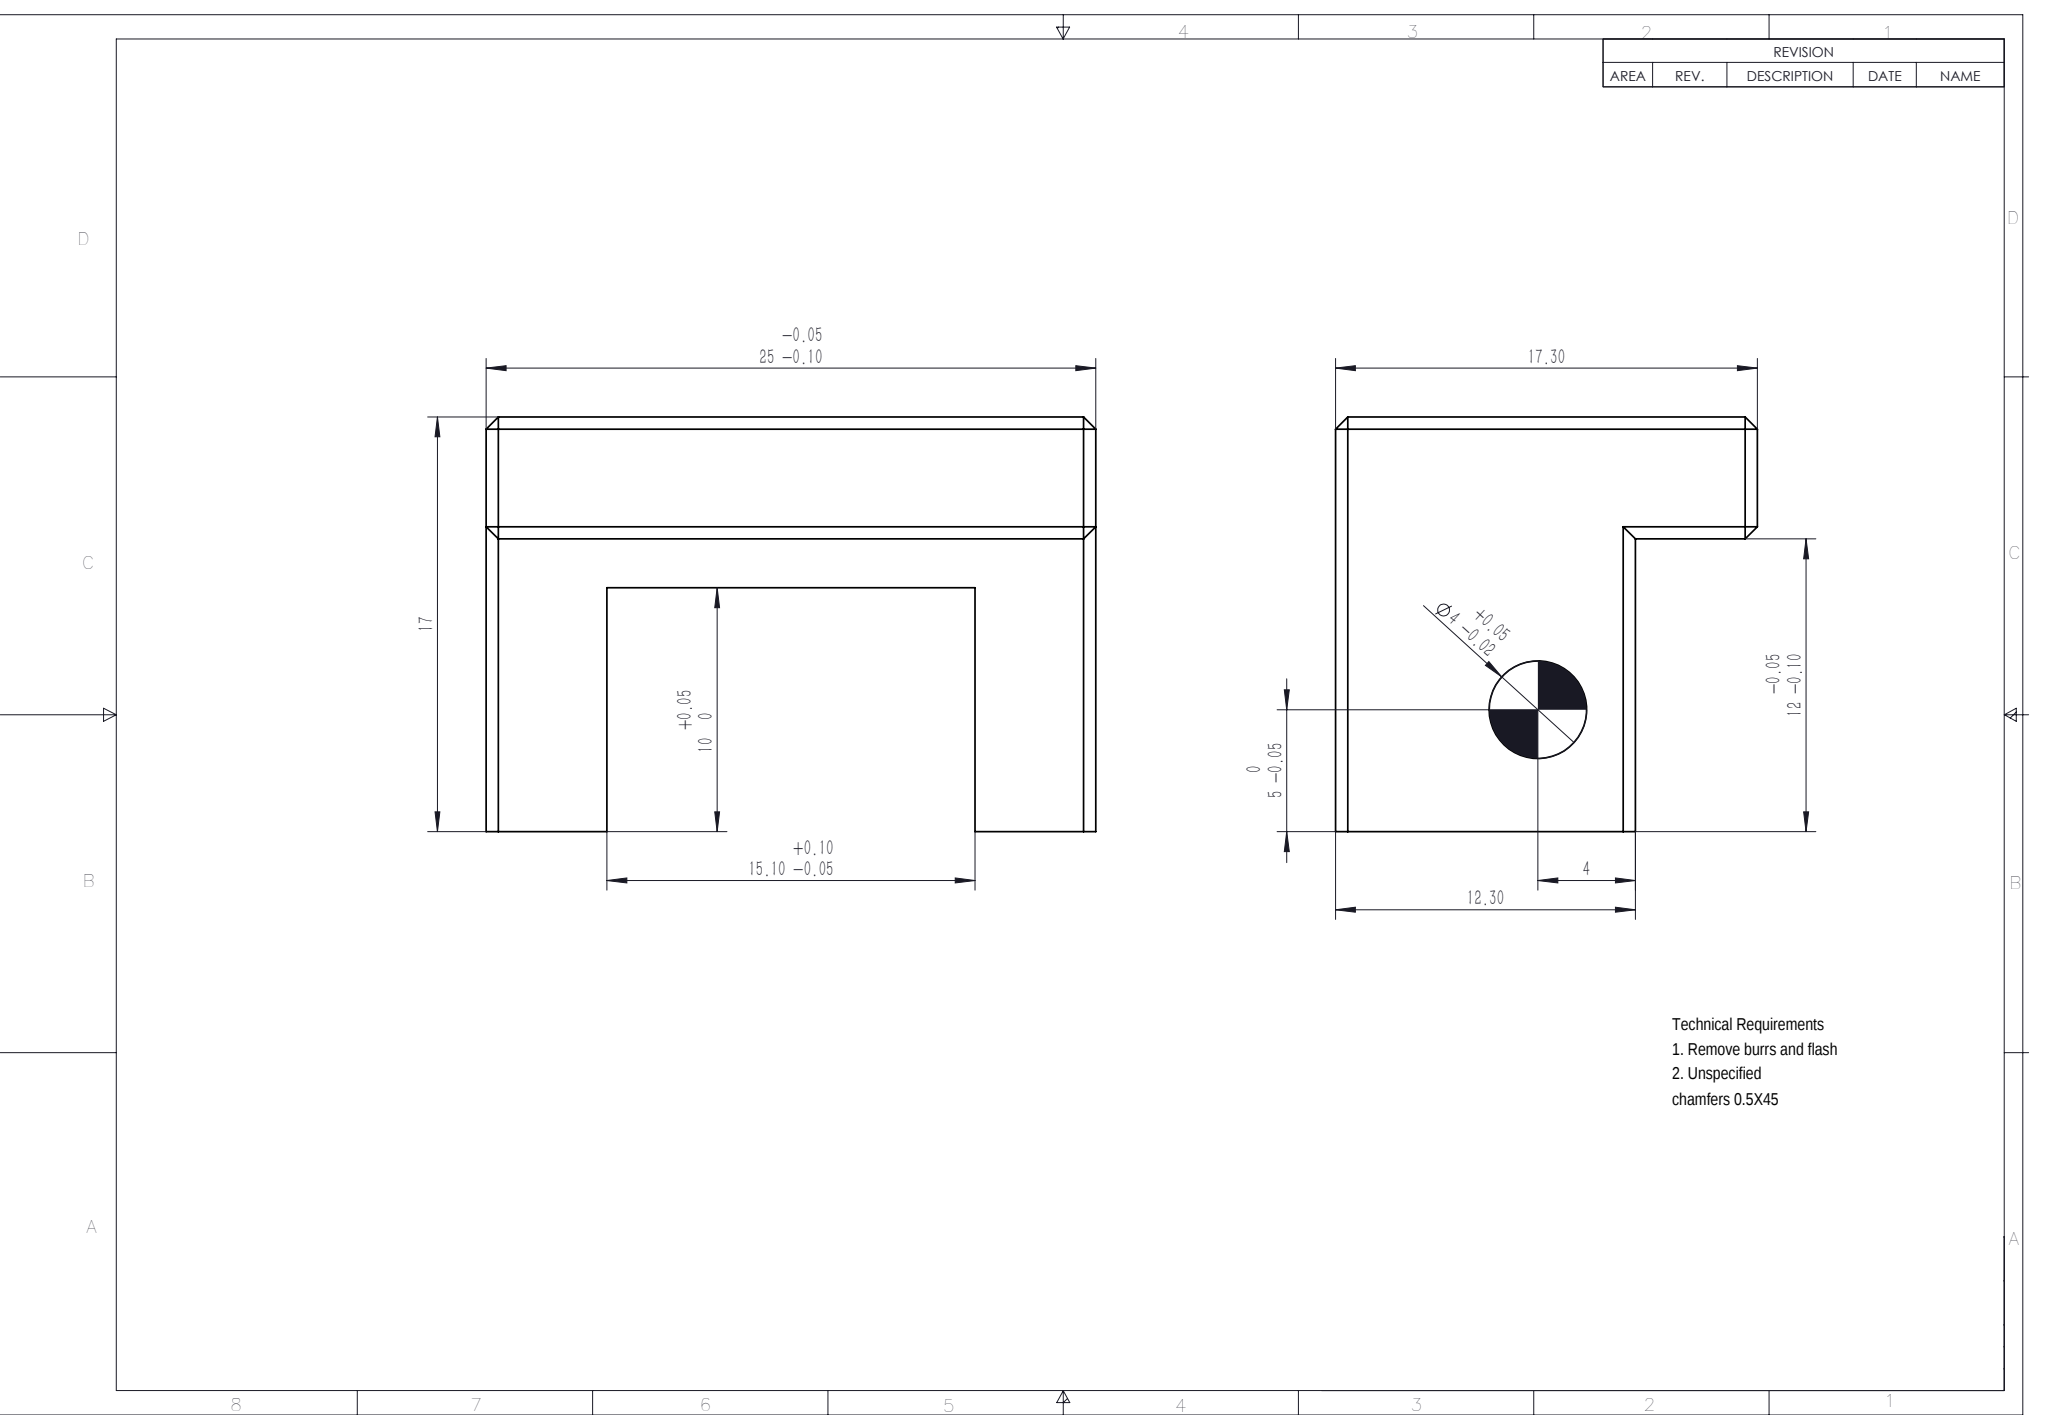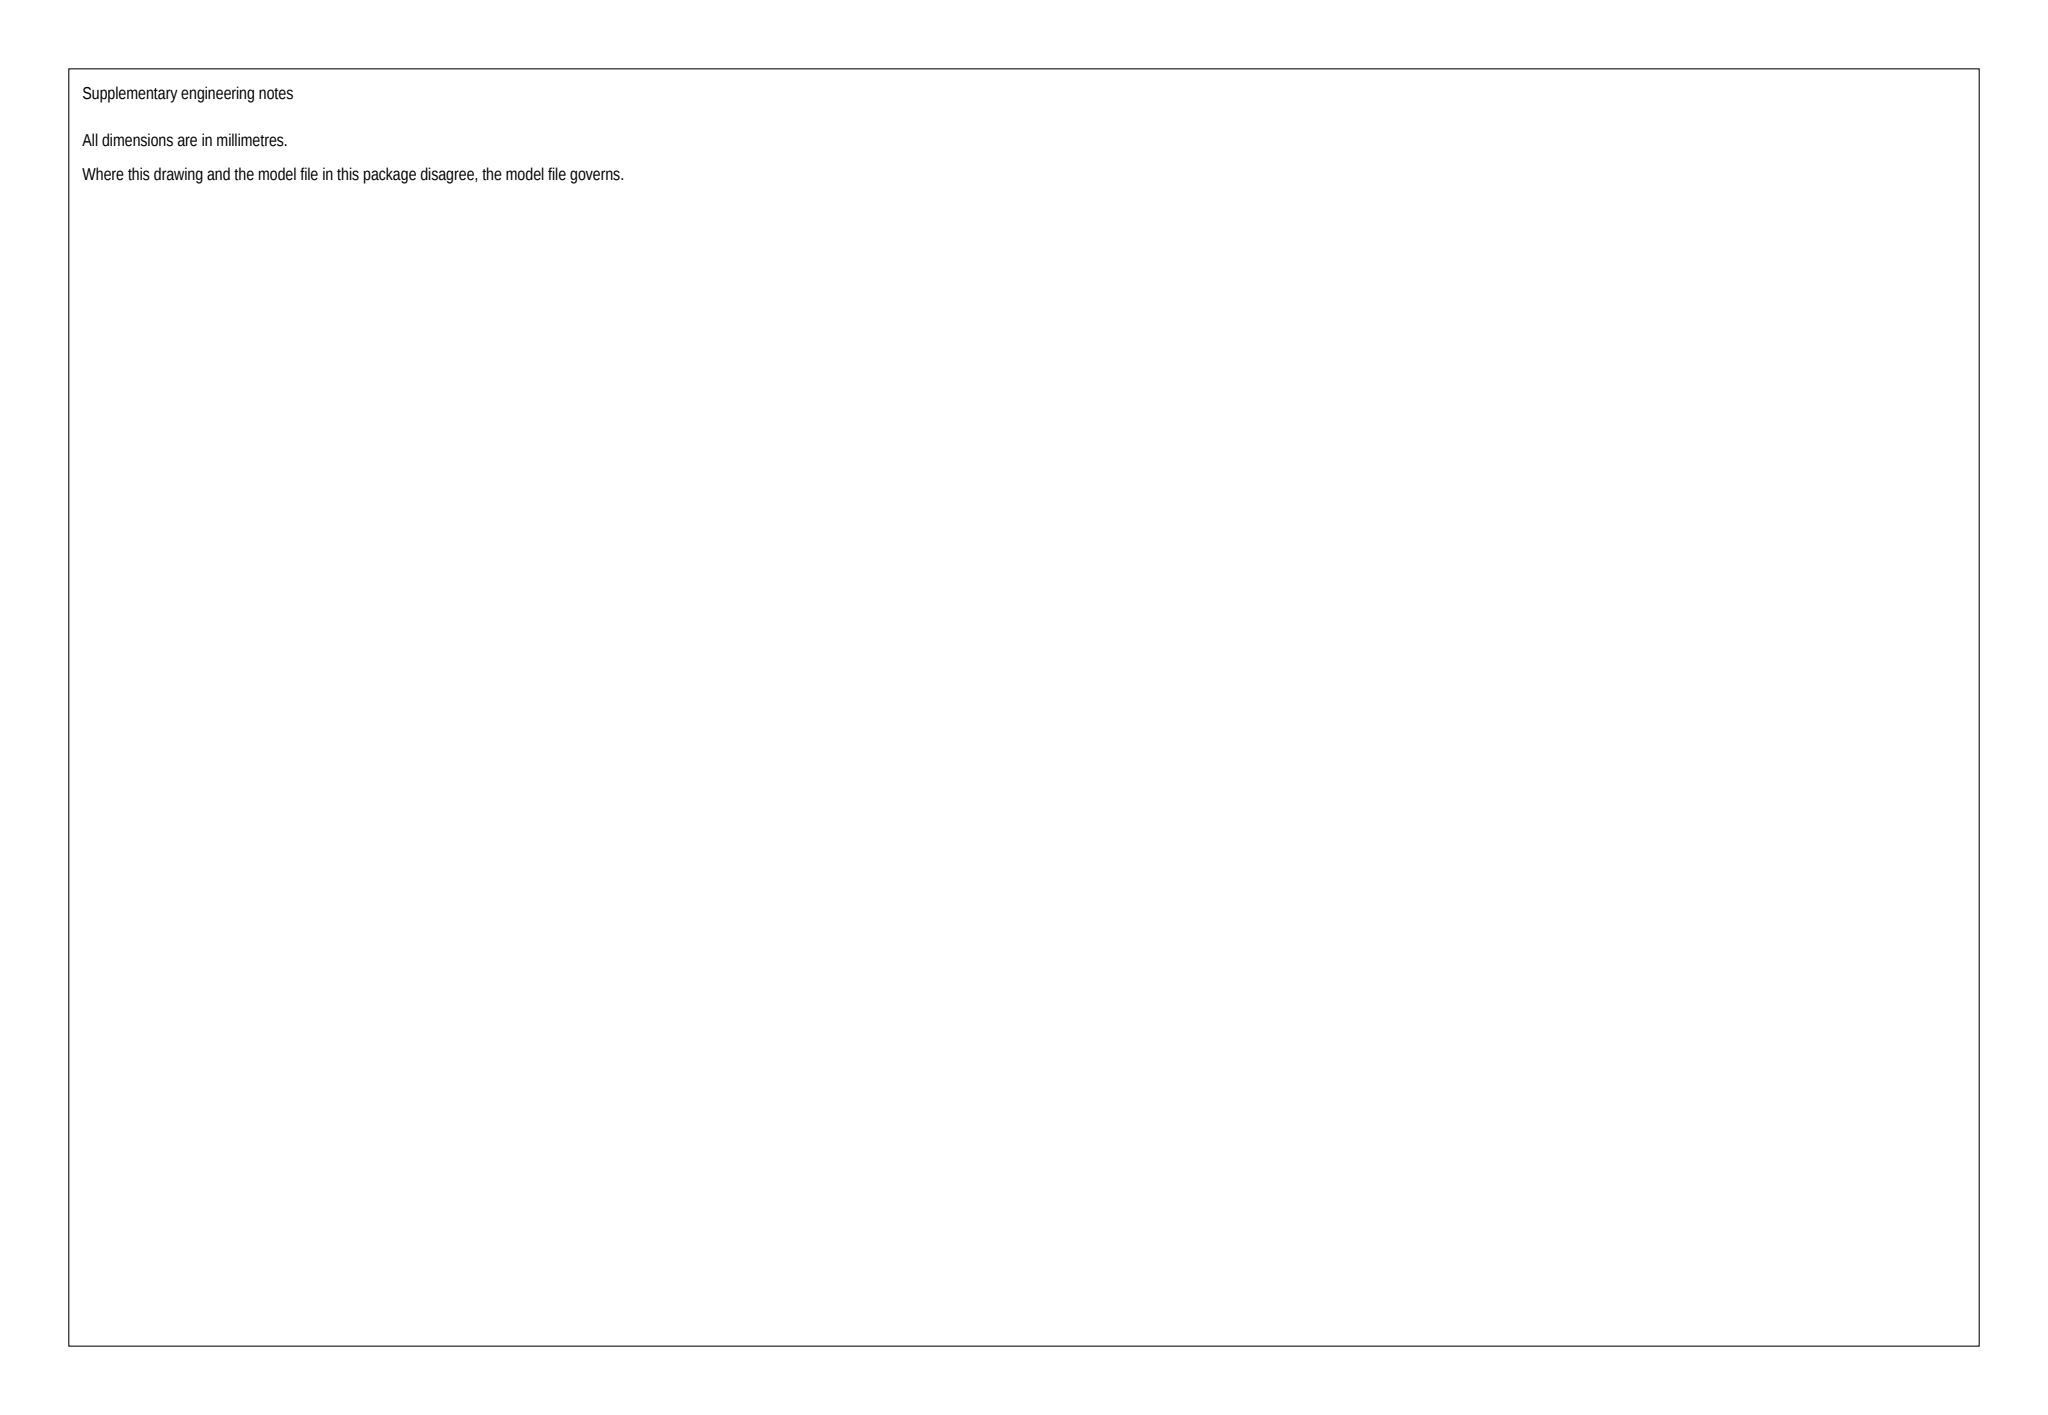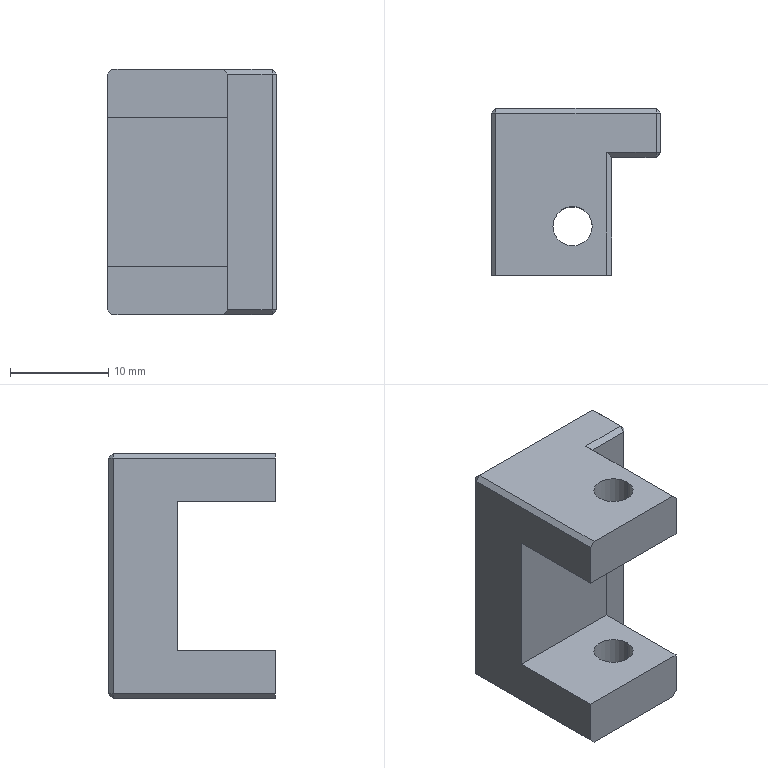Part | SolidWorks | 1 solid | 35 faces | box 17.3 x 17 x 25 mm | volume 3848 mm3 | plane 31 | cylinder 4 | commonest cylinder face diameters 4 x4
build123d program:
from build123d import *

# Parameters (mm, degrees)
SKETCH1_W                      = 12.3
SKETCH1_H                      = 25
BOSS_EXTRUDE1_DEPTH            = 88
SKETCH2_W                      = 25
SKETCH2_H                      = 5
BOSS_EXTRUDE2_DEPTH            = 5
SKETCH4_W                      = 15
SKETCH4_H                      = 35
CUT_EXTRUDE1_DEPTH             = 90.73
SIZE_MM_DOWEL_PIN_HOLE_1_D     = 4
SKETCH7_W                      = 12.3
SKETCH7_H                      = 10
CUT_EXTRUDE2_DEPTH             = 93.159
F_4_0_4_DIAMETER_HOLE1_D       = 8
F_4_0_4_DIAMETER_HOLE1_DEPTH   = 5
SKETCH11_W                     = 12.3
SKETCH11_H                     = 61
CUT_EXTRUDE4_DEPTH             = 93.159
SKETCH12_W                     = 15.1
SKETCH12_H                     = 10
CUT_EXTRUDE5_DEPTH             = 90.73
SIZE_MM_DOWEL_PIN_HOLE_2_D     = 4
SIZE_MM_DOWEL_PIN_HOLE_2_DEPTH = 35
CHAMFER1_SIZE                  = 0.5


with BuildPart() as part:
    # Sketch1 → Boss-Extrude1 (new body)
    with BuildSketch(Plane(origin=(0, 0, 0), x_dir=(1, 0, 0), z_dir=(0, 1, 0))):
        Rectangle(SKETCH1_W, SKETCH1_H)
    extrude(amount=BOSS_EXTRUDE1_DEPTH)

    # Sketch2 → Boss-Extrude2 (add)
    with BuildSketch(Plane(origin=(6.15, 0, 0), x_dir=(0, 0, -1), z_dir=(1, 0, 0))):
        with Locations((0, 85.5)):
            Rectangle(SKETCH2_W, SKETCH2_H)
    extrude(amount=BOSS_EXTRUDE2_DEPTH)

    # Sketch4 → Cut-Extrude1 (cut, through all)
    with BuildSketch(Plane(origin=(6.15, 0, 0), x_dir=(0, 0, -1), z_dir=(1, 0, 0))):
        with Locations((0, 17.5)):
            Rectangle(SKETCH4_W, SKETCH4_H)
    extrude(amount=-CUT_EXTRUDE1_DEPTH, mode=Mode.SUBTRACT)

    # Size mm Dowel Pin Hole 1 (through all)
    with Locations(Plane(origin=(0, 0, -12.5), x_dir=(-1, 0, 0), z_dir=(0, 0, -1))):
        with Locations((1.15, 30), (1.15, 15)):
            Hole(SIZE_MM_DOWEL_PIN_HOLE_1_D / 2)

    # Sketch7 → Cut-Extrude2 (cut, through all)
    with BuildSketch(Plane.XY.offset(12.5)):
        with Locations((0, 5)):
            Rectangle(SKETCH7_W, SKETCH7_H)
    extrude(amount=-CUT_EXTRUDE2_DEPTH, mode=Mode.SUBTRACT)

    # 4.0 _4_ Diameter Hole1
    with Locations(Plane(origin=(6.15, 0, 0), x_dir=(0, 0, -1), z_dir=(1, 0, 0))):
        with Locations((-7.5, 58), (7.5, 58)):
            Hole(F_4_0_4_DIAMETER_HOLE1_D / 2, depth=F_4_0_4_DIAMETER_HOLE1_DEPTH)

    # Sketch11 → Cut-Extrude4 (cut, through all)
    with BuildSketch(Plane(origin=(0, 0, -12.5), x_dir=(-1, 0, 0), z_dir=(0, 0, -1))):
        with Locations((0, 40.5)):
            Rectangle(SKETCH11_W, SKETCH11_H)
    extrude(amount=-CUT_EXTRUDE4_DEPTH, mode=Mode.SUBTRACT)

    # Sketch12 → Cut-Extrude5 (cut, through all)
    with BuildSketch(Plane(origin=(6.15, 0, 0), x_dir=(0, 0, -1), z_dir=(1, 0, 0))):
        with Locations((0, 76)):
            Rectangle(SKETCH12_W, SKETCH12_H)
    extrude(amount=-CUT_EXTRUDE5_DEPTH, mode=Mode.SUBTRACT)

    # Size mm Dowel Pin Hole 2
    with Locations(Plane(origin=(0, 0, -12.5), x_dir=(-1, 0, 0), z_dir=(0, 0, -1))):
        with Locations((-2.15, 76)):
            Hole(SIZE_MM_DOWEL_PIN_HOLE_2_D / 2, depth=SIZE_MM_DOWEL_PIN_HOLE_2_DEPTH)

    # Chamfer1
    chamfer1_edges = [part.edges().sort_by_distance(p)[0] for p in [
        (-6.15, 88, 0),
        (11.15, 88, 0),
        (-6.15, 79.5, 12.5),
        (2.5, 88, 12.5),
        (6.15, 77, -12.5),
        (8.65, 83, -12.5),
        (6.15, 77, 12.5),
        (8.65, 83, 12.5),
        (11.15, 85.5, 12.5),
        (11.15, 83, 0),
        (11.15, 85.5, -12.5),
        (2.5, 88, -12.5),
        (-6.15, 79.5, -12.5),
    ]]
    chamfer(chamfer1_edges, length=CHAMFER1_SIZE)


solid = part.part